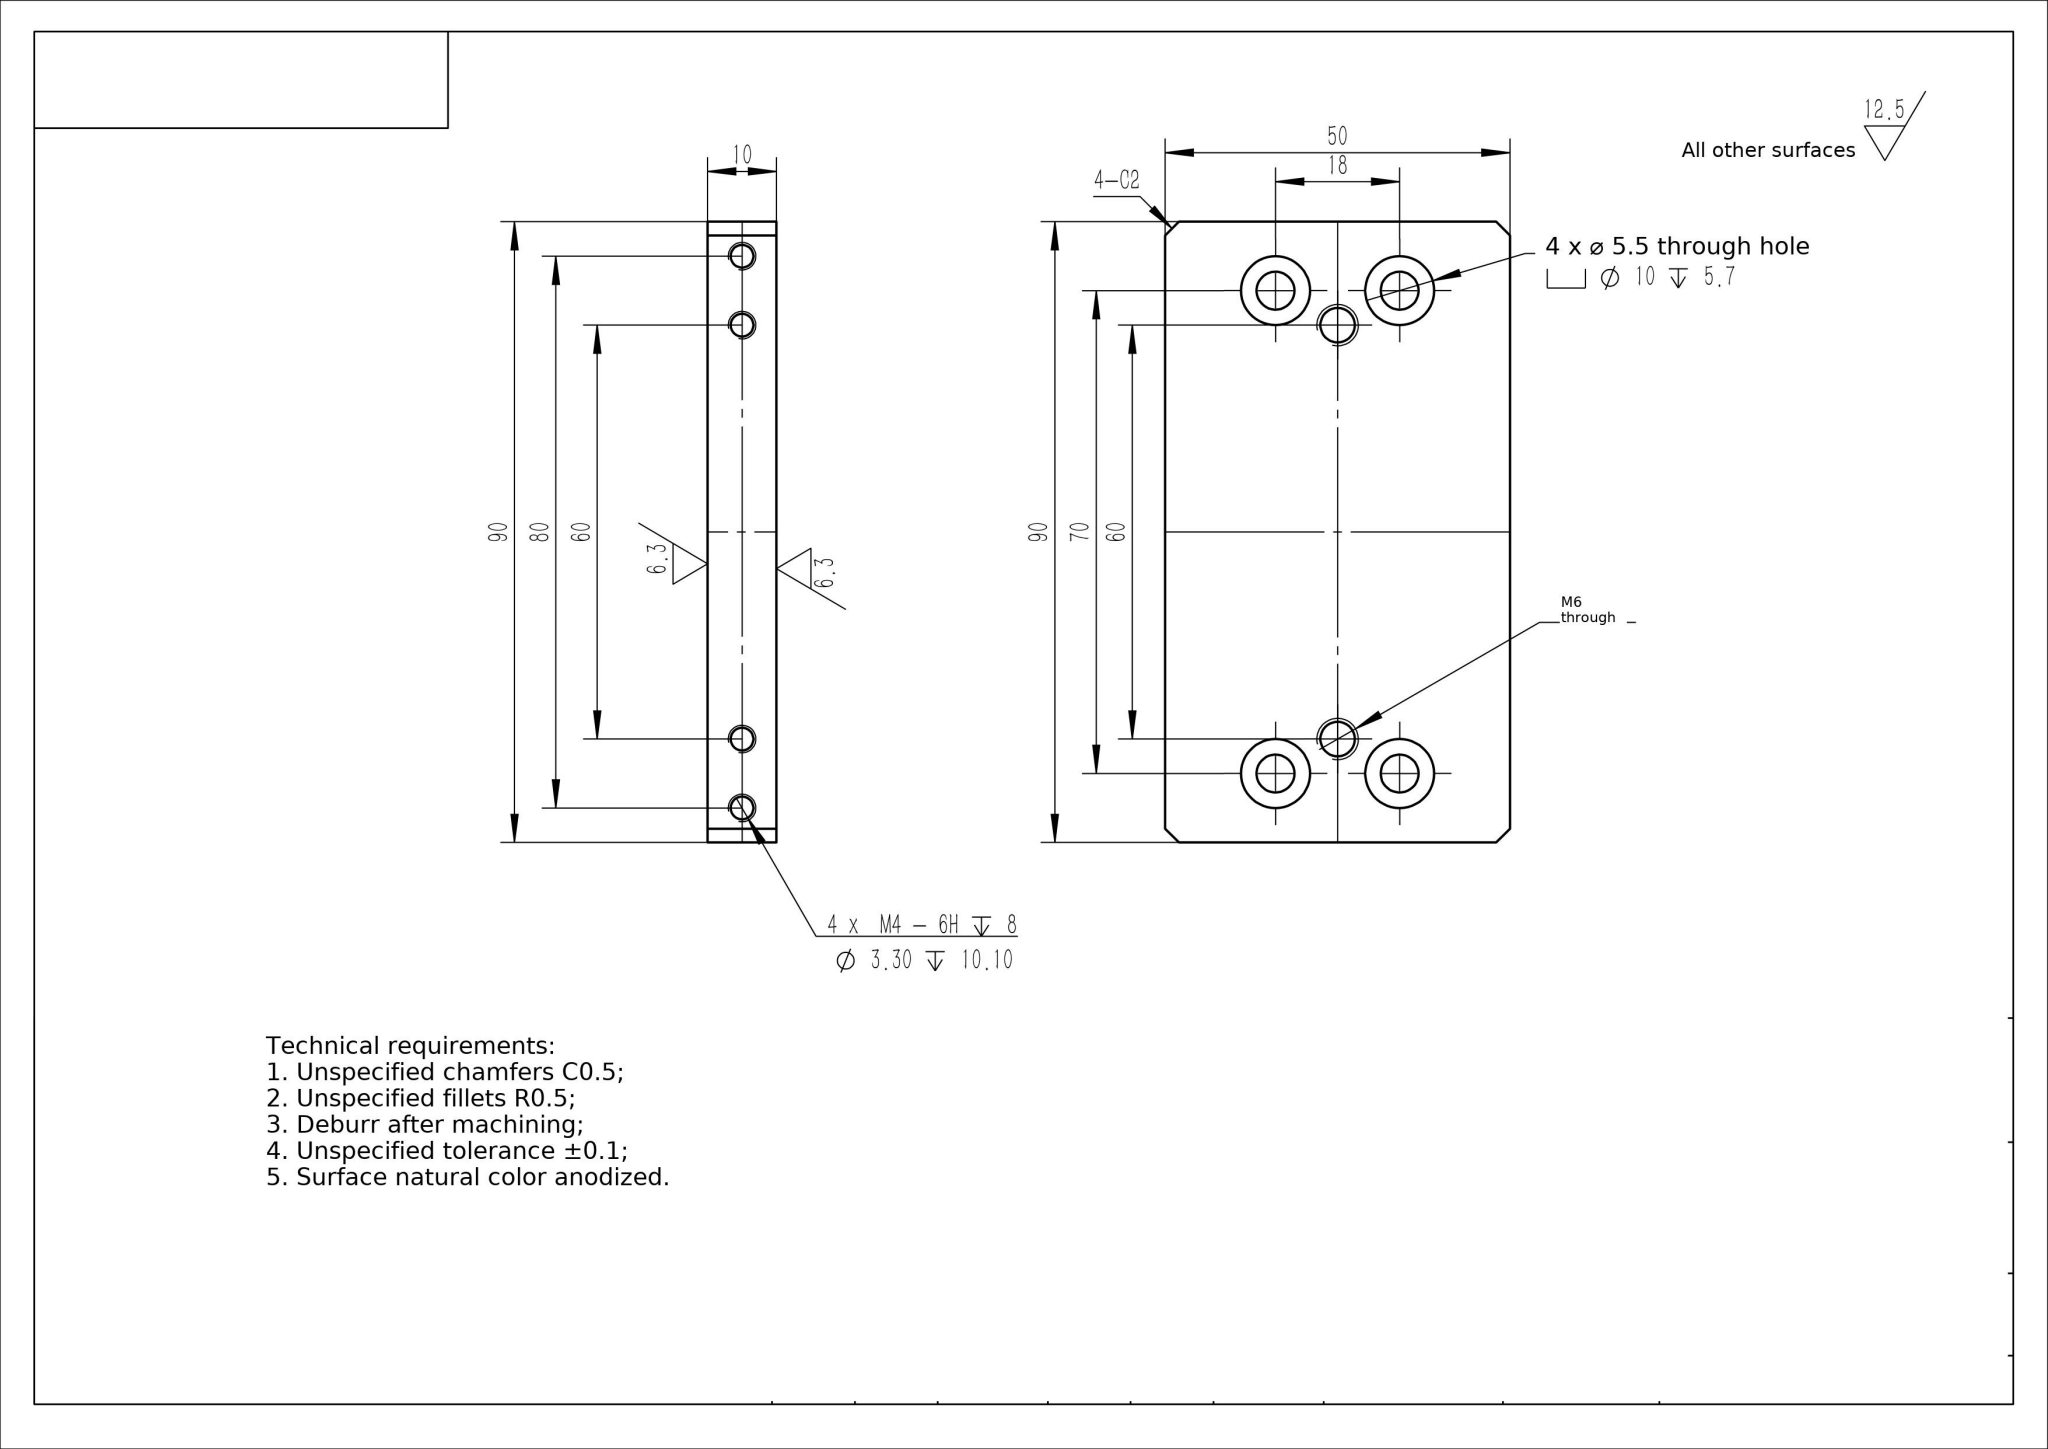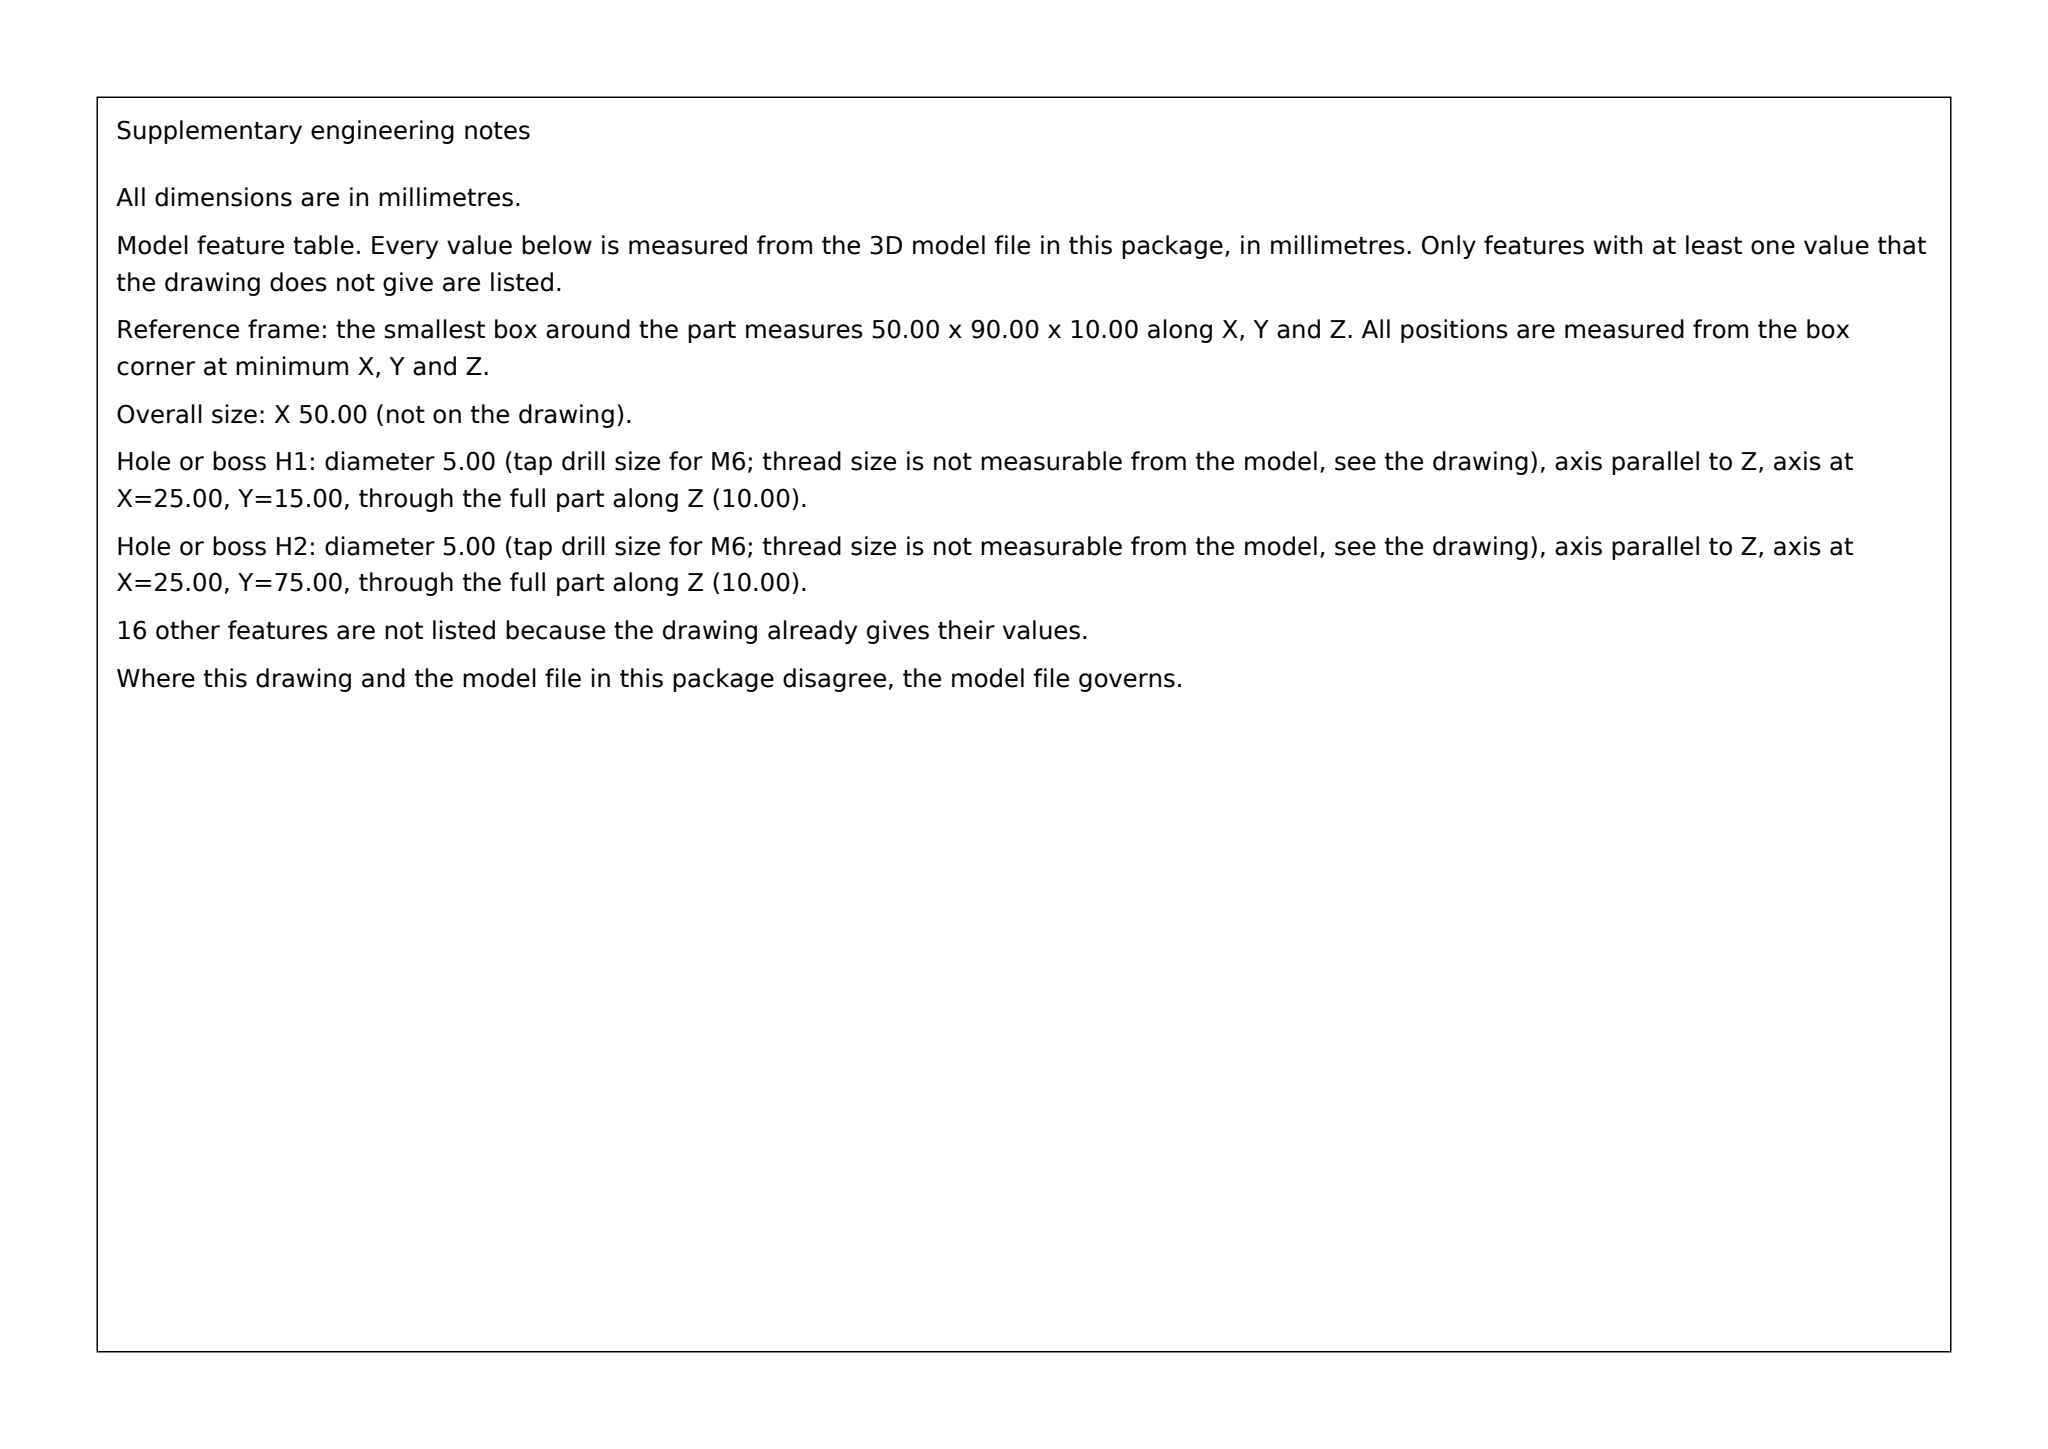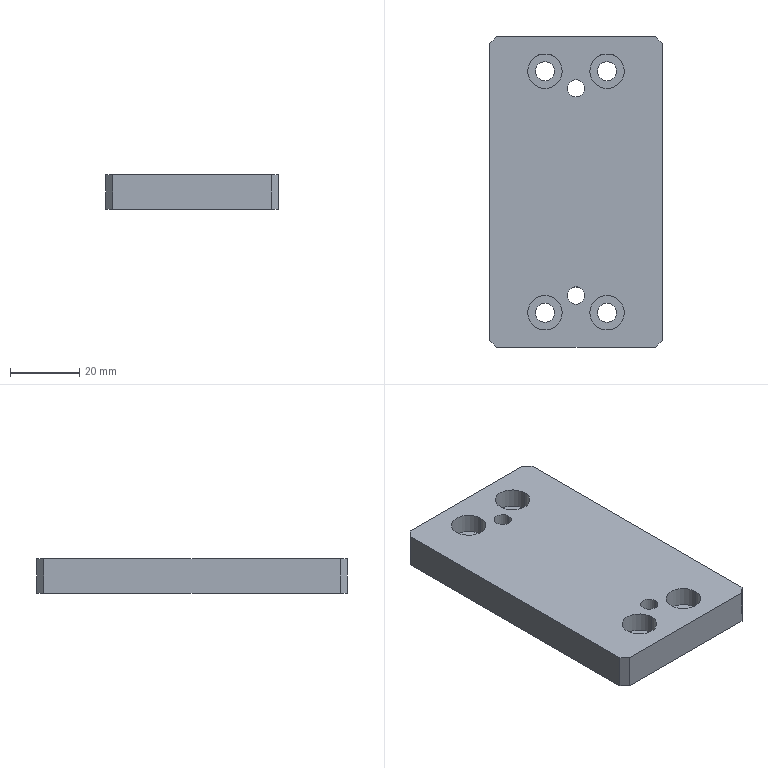Part | SolidWorks | mm | 1 solid | 50 faces | box 50 x 90 x 10 mm | volume 41971 mm3 | cylinder 28 | plane 14 | cone 8 | commonest cylinder face diameters 3.3 x8 10 x8 5.5 x8 5 x4
build123d program:
from build123d import *

# Parameters (mm, degrees)
SKETCH1_W                                         = 50
SKETCH1_H                                         = 90
BOSS_EXTRUDE1_DEPTH                               = 10
M6_TAPPED_HOLE1_D                                 = 5
CHAMFER1_SIZE                                     = 2
HOLE_SIZE_ACCORDING_TO_HEXAGON_SOCKET_D           = 5.5
HOLE_SIZE_ACCORDING_TO_HEXAGON_SOCKET_CBORE_D     = 10
HOLE_SIZE_ACCORDING_TO_HEXAGON_SOCKET_CBORE_DEPTH = 5.7
M4_TAPPED_HOLE1_D                                 = 3.3
M4_TAPPED_HOLE1_DEPTH                             = 10.1
M4_TAPPED_HOLE1_TIP                               = 0.9914


with BuildPart() as part:
    # Sketch1 → Boss-Extrude1 (new body)
    with BuildSketch(Plane.XY):
        Rectangle(SKETCH1_W, SKETCH1_H)
    extrude(amount=BOSS_EXTRUDE1_DEPTH)

    # M6 Tapped Hole1 (through all)
    with Locations(Plane.XY.offset(10)):
        with Locations((0, 30), (0, -30)):
            Hole(M6_TAPPED_HOLE1_D / 2)

    # Chamfer1
    chamfer1_edges = [part.edges().sort_by_distance(p)[0] for p in [
        (-25, 45, 5),
        (25, 45, 5),
        (25, -45, 5),
        (-25, -45, 5),
    ]]
    chamfer(chamfer1_edges, length=CHAMFER1_SIZE)

    # Hole Size _ according to_ Hexagon socket (through all)
    with Locations(Plane.XY.offset(10)):
        with Locations((-9, 35), (-9, -35), (9, -35), (9, 35)):
            CounterBoreHole(HOLE_SIZE_ACCORDING_TO_HEXAGON_SOCKET_D / 2, HOLE_SIZE_ACCORDING_TO_HEXAGON_SOCKET_CBORE_D / 2, HOLE_SIZE_ACCORDING_TO_HEXAGON_SOCKET_CBORE_DEPTH)

    # M4 Tapped Hole1
    with Locations(Plane(origin=(25, 0, 0), x_dir=(0, 0, -1), z_dir=(1, 0, 0))):
        with Locations((-5, 30), (-5, 40), (-5, -40), (-5, -30)):
            Hole(M4_TAPPED_HOLE1_D / 2, depth=M4_TAPPED_HOLE1_DEPTH)
            with Locations((0, 0, -(M4_TAPPED_HOLE1_DEPTH + M4_TAPPED_HOLE1_TIP / 2))):  # 118° drill point
                Cone(0, M4_TAPPED_HOLE1_D / 2, M4_TAPPED_HOLE1_TIP, mode=Mode.SUBTRACT)


solid = part.part